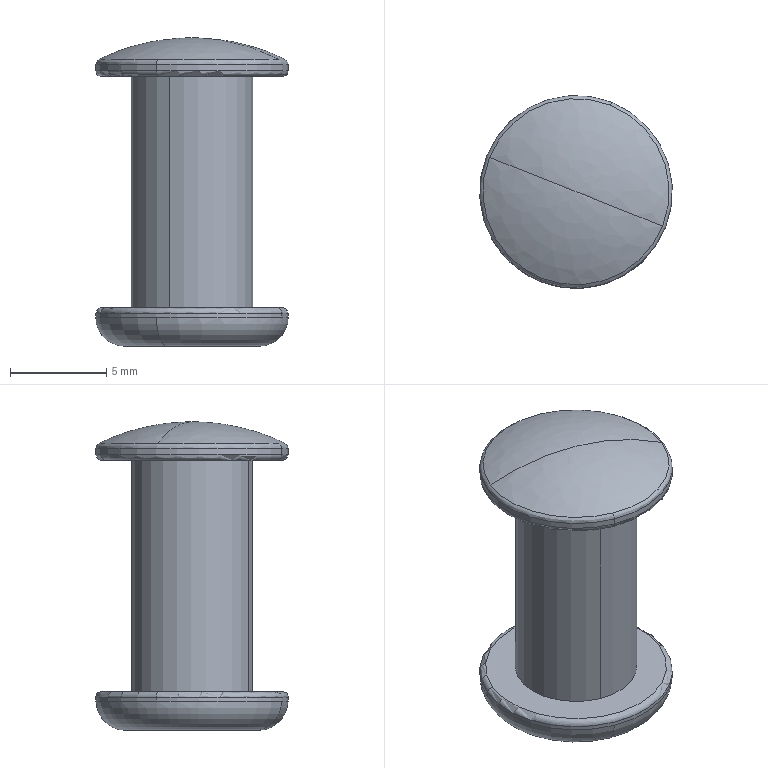Component | SolidWorks | CH-225-D-1_225-D-05-1 | 1 solid | 23 faces | box 10 x 10 x 16 mm | volume 564 mm3 | cylinder 8 | torus 6 | spline 4 | plane 3 | cone 2 | commonest cylinder face diameters 10 x4 6.3 x2 4.833 x2
STEP:
#1=COLOUR_RGB('',0.7922,0.8196,0.9333);
#2=FILL_AREA_STYLE_COLOUR('',#1);
#3=FILL_AREA_STYLE('',(#2));
#4=SURFACE_STYLE_FILL_AREA(#3);
#5=SURFACE_SIDE_STYLE('',(#4));
#6=SURFACE_STYLE_USAGE(.BOTH.,#5);
#7=PRESENTATION_STYLE_ASSIGNMENT((#6));
#8=CARTESIAN_POINT('',(0.9006,3.358,4.958));
#9=VERTEX_POINT('',#8);
#10=CARTESIAN_POINT('',(1.077,3.288,4.914));
#11=VERTEX_POINT('',#10);
#12=CARTESIAN_POINT('',(0.9006,3.358,4.525));
#13=DIRECTION('',(0.3691,0.9294,0.));
#14=DIRECTION('',(0.,0.,1.));
#15=AXIS2_PLACEMENT_3D('',#12,#13,#14);
#16=CIRCLE('',#15,0.4332);
#17=EDGE_CURVE('',#9,#11,#16,.T.);
#18=ORIENTED_EDGE('',*,*,#17,.F.);
#19=CARTESIAN_POINT('',(0.7238,3.429,4.914));
#20=VERTEX_POINT('',#19);
#21=CARTESIAN_POINT('',(0.9006,3.358,4.525));
#22=DIRECTION('',(-0.3691,-0.9294,0.));
#23=DIRECTION('',(0.,0.,1.));
#24=AXIS2_PLACEMENT_3D('',#21,#22,#23);
#25=CIRCLE('',#24,0.4332);
#26=EDGE_CURVE('',#9,#20,#25,.T.);
#27=ORIENTED_EDGE('',*,*,#26,.T.);
#28=CARTESIAN_POINT('',(0.8304,3.182,4.914));
#29=VERTEX_POINT('',#28);
#30=CARTESIAN_POINT('',(0.9006,3.358,4.914));
#31=DIRECTION('',(0.,0.,-1.));
#32=DIRECTION('',(0.3691,0.9294,0.));
#33=AXIS2_PLACEMENT_3D('',#30,#31,#32);
#34=CIRCLE('',#33,0.1902);
#35=EDGE_CURVE('',#29,#20,#34,.T.);
#36=ORIENTED_EDGE('',*,*,#35,.F.);
#37=CARTESIAN_POINT('',(0.9006,3.358,4.914));
#38=DIRECTION('',(0.,0.,-1.));
#39=DIRECTION('',(0.3691,0.9294,0.));
#40=AXIS2_PLACEMENT_3D('',#37,#38,#39);
#41=CIRCLE('',#40,0.1902);
#42=EDGE_CURVE('',#11,#29,#41,.T.);
#43=ORIENTED_EDGE('',*,*,#42,.F.);
#44=EDGE_LOOP('',(#18,#27,#36,#43));
#45=FACE_OUTER_BOUND('',#44,.T.);
#46=CARTESIAN_POINT('',(0.9006,3.358,4.958));
#47=CARTESIAN_POINT('',(0.9006,3.358,4.958));
#48=CARTESIAN_POINT('',(0.9006,3.358,4.958));
#49=CARTESIAN_POINT('',(0.9006,3.358,4.958));
#50=CARTESIAN_POINT('',(0.9622,3.334,4.958));
#51=CARTESIAN_POINT('',(0.9133,3.211,4.958));
#52=CARTESIAN_POINT('',(0.7902,3.26,4.958));
#53=CARTESIAN_POINT('',(0.8391,3.383,4.958));
#54=CARTESIAN_POINT('',(1.022,3.31,4.943));
#55=CARTESIAN_POINT('',(0.9256,3.067,4.943));
#56=CARTESIAN_POINT('',(0.6826,3.164,4.943));
#57=CARTESIAN_POINT('',(0.7791,3.407,4.943));
#58=CARTESIAN_POINT('',(1.077,3.288,4.914));
#59=CARTESIAN_POINT('',(0.937,2.935,4.914));
#60=CARTESIAN_POINT('',(0.5834,3.075,4.914));
#61=CARTESIAN_POINT('',(0.7238,3.429,4.914));
#62=(BOUNDED_SURFACE()B_SPLINE_SURFACE(3,3,((#46,#47,#48,#49),(#50,#51,#52,#53),(#54,#55,#56,#57),(#58,#59,#60,#61)),.UNSPECIFIED.,.F.,.F.,.F.)B_SPLINE_SURFACE_WITH_KNOTS((4,4),(4,4),(0.,1.),(0.,1.),.UNSPECIFIED.)GEOMETRIC_REPRESENTATION_ITEM()RATIONAL_B_SPLINE_SURFACE(((1.,0.3333,0.3333,1.),(0.9829,0.3276,0.3276,0.9829),(0.9829,0.3276,0.3276,0.9829),(1.,0.3333,0.3333,1.)))REPRESENTATION_ITEM('')SURFACE());
#63=ADVANCED_FACE('',(#45),#62,.F.);
#64=CARTESIAN_POINT('',(0.8548,3.243,4.879));
#65=VERTEX_POINT('',#64);
#66=CARTESIAN_POINT('',(0.9464,3.474,4.879));
#67=VERTEX_POINT('',#66);
#68=CARTESIAN_POINT('',(0.9006,3.358,4.879));
#69=DIRECTION('',(0.,0.,1.));
#70=DIRECTION('',(0.3691,0.9294,0.));
#71=AXIS2_PLACEMENT_3D('',#68,#69,#70);
#72=CIRCLE('',#71,0.124);
#73=EDGE_CURVE('',#65,#67,#72,.T.);
#74=ORIENTED_EDGE('',*,*,#73,.F.);
#75=CARTESIAN_POINT('',(0.8548,3.243,4.407));
#76=VERTEX_POINT('',#75);
#77=CARTESIAN_POINT('',(0.8548,3.243,4.879));
#78=DIRECTION('',(0.,0.,-1.));
#79=VECTOR('',#78,39.37);
#80=LINE('',#77,#79);
#81=EDGE_CURVE('',#65,#76,#80,.T.);
#82=ORIENTED_EDGE('',*,*,#81,.T.);
#83=CARTESIAN_POINT('',(0.9464,3.474,4.407));
#84=VERTEX_POINT('',#83);
#85=CARTESIAN_POINT('',(0.9006,3.358,4.407));
#86=DIRECTION('',(0.,0.,-1.));
#87=DIRECTION('',(0.3691,0.9294,0.));
#88=AXIS2_PLACEMENT_3D('',#85,#86,#87);
#89=CIRCLE('',#88,0.124);
#90=EDGE_CURVE('',#84,#76,#89,.T.);
#91=ORIENTED_EDGE('',*,*,#90,.F.);
#92=CARTESIAN_POINT('',(0.9464,3.474,4.879));
#93=DIRECTION('',(0.,0.,-1.));
#94=VECTOR('',#93,39.37);
#95=LINE('',#92,#94);
#96=EDGE_CURVE('',#67,#84,#95,.T.);
#97=ORIENTED_EDGE('',*,*,#96,.F.);
#98=EDGE_LOOP('',(#74,#82,#91,#97));
#99=FACE_OUTER_BOUND('',#98,.T.);
#100=CARTESIAN_POINT('',(0.9006,3.358,4.879));
#101=DIRECTION('',(0.,0.,-1.));
#102=DIRECTION('',(0.3691,0.9294,0.));
#103=AXIS2_PLACEMENT_3D('',#100,#101,#102);
#104=CYLINDRICAL_SURFACE('',#103,0.124);
#105=ADVANCED_FACE('',(#99),#104,.T.);
#106=CARTESIAN_POINT('',(0.9733,3.541,4.891));
#107=VERTEX_POINT('',#106);
#108=CARTESIAN_POINT('',(0.828,3.175,4.891));
#109=VERTEX_POINT('',#108);
#110=CARTESIAN_POINT('',(0.9006,3.358,4.891));
#111=DIRECTION('',(0.,0.,-1.));
#112=DIRECTION('',(0.3691,0.9294,0.));
#113=AXIS2_PLACEMENT_3D('',#110,#111,#112);
#114=CIRCLE('',#113,0.1969);
#115=EDGE_CURVE('',#107,#109,#114,.T.);
#116=ORIENTED_EDGE('',*,*,#115,.T.);
#117=CARTESIAN_POINT('',(0.8323,3.186,4.879));
#118=VERTEX_POINT('',#117);
#119=CARTESIAN_POINT('',(0.8323,3.186,4.891));
#120=DIRECTION('',(0.9294,-0.3691,0.));
#121=DIRECTION('',(0.3691,0.9294,0.));
#122=AXIS2_PLACEMENT_3D('',#119,#120,#121);
#123=CIRCLE('',#122,0.01181);
#124=EDGE_CURVE('',#109,#118,#123,.T.);
#125=ORIENTED_EDGE('',*,*,#124,.T.);
#126=CARTESIAN_POINT('',(0.9689,3.53,4.879));
#127=VERTEX_POINT('',#126);
#128=CARTESIAN_POINT('',(0.9006,3.358,4.879));
#129=DIRECTION('',(0.,0.,1.));
#130=DIRECTION('',(0.3691,0.9294,0.));
#131=AXIS2_PLACEMENT_3D('',#128,#129,#130);
#132=CIRCLE('',#131,0.185);
#133=EDGE_CURVE('',#118,#127,#132,.T.);
#134=ORIENTED_EDGE('',*,*,#133,.T.);
#135=CARTESIAN_POINT('',(0.9689,3.53,4.891));
#136=DIRECTION('',(-0.9294,0.3691,0.));
#137=DIRECTION('',(-0.3691,-0.9294,0.));
#138=AXIS2_PLACEMENT_3D('',#135,#136,#137);
#139=CIRCLE('',#138,0.01181);
#140=EDGE_CURVE('',#107,#127,#139,.T.);
#141=ORIENTED_EDGE('',*,*,#140,.F.);
#142=EDGE_LOOP('',(#116,#125,#134,#141));
#143=FACE_OUTER_BOUND('',#142,.T.);
#144=CARTESIAN_POINT('',(0.9006,3.358,4.891));
#145=DIRECTION('',(0.,0.,-1.));
#146=DIRECTION('',(0.3691,0.9294,0.));
#147=AXIS2_PLACEMENT_3D('',#144,#145,#146);
#148=TOROIDAL_SURFACE('',#147,0.185,0.01181);
#149=ADVANCED_FACE('',(#143),#148,.T.);
#150=CARTESIAN_POINT('',(0.7286,3.427,4.407));
#151=VERTEX_POINT('',#150);
#152=CARTESIAN_POINT('',(1.073,3.29,4.407));
#153=VERTEX_POINT('',#152);
#154=CARTESIAN_POINT('',(0.9006,3.358,4.407));
#155=DIRECTION('',(0.,-0.,-1.));
#156=DIRECTION('',(-0.9294,0.3691,0.));
#157=AXIS2_PLACEMENT_3D('',#154,#155,#156);
#158=CIRCLE('',#157,0.185);
#159=EDGE_CURVE('',#151,#153,#158,.T.);
#160=ORIENTED_EDGE('',*,*,#159,.T.);
#161=CARTESIAN_POINT('',(1.084,3.286,4.395));
#162=VERTEX_POINT('',#161);
#163=CARTESIAN_POINT('',(1.073,3.29,4.395));
#164=DIRECTION('',(0.3691,0.9294,-0.));
#165=DIRECTION('',(-0.9294,0.3691,0.));
#166=AXIS2_PLACEMENT_3D('',#163,#164,#165);
#167=CIRCLE('',#166,0.01181);
#168=EDGE_CURVE('',#153,#162,#167,.T.);
#169=ORIENTED_EDGE('',*,*,#168,.T.);
#170=CARTESIAN_POINT('',(0.7177,3.431,4.395));
#171=VERTEX_POINT('',#170);
#172=CARTESIAN_POINT('',(0.9006,3.358,4.395));
#173=DIRECTION('',(-0.,0.,1.));
#174=DIRECTION('',(0.9294,-0.3691,0.));
#175=AXIS2_PLACEMENT_3D('',#172,#173,#174);
#176=CIRCLE('',#175,0.1969);
#177=EDGE_CURVE('',#162,#171,#176,.T.);
#178=ORIENTED_EDGE('',*,*,#177,.T.);
#179=CARTESIAN_POINT('',(0.7286,3.427,4.395));
#180=DIRECTION('',(-0.3691,-0.9294,0.));
#181=DIRECTION('',(0.9294,-0.3691,0.));
#182=AXIS2_PLACEMENT_3D('',#179,#180,#181);
#183=CIRCLE('',#182,0.01181);
#184=EDGE_CURVE('',#151,#171,#183,.T.);
#185=ORIENTED_EDGE('',*,*,#184,.F.);
#186=EDGE_LOOP('',(#160,#169,#178,#185));
#187=FACE_OUTER_BOUND('',#186,.T.);
#188=CARTESIAN_POINT('',(0.9006,3.358,4.395));
#189=DIRECTION('',(0.,-0.,-1.));
#190=DIRECTION('',(-0.9294,0.3691,-0.));
#191=AXIS2_PLACEMENT_3D('',#188,#189,#190);
#192=TOROIDAL_SURFACE('',#191,0.185,0.01181);
#193=ADVANCED_FACE('',(#187),#192,.T.);
#194=CARTESIAN_POINT('',(0.828,3.175,4.903));
#195=VERTEX_POINT('',#194);
#196=CARTESIAN_POINT('',(0.9733,3.541,4.903));
#197=VERTEX_POINT('',#196);
#198=CARTESIAN_POINT('',(0.9006,3.358,4.903));
#199=DIRECTION('',(0.,0.,1.));
#200=DIRECTION('',(0.3691,0.9294,0.));
#201=AXIS2_PLACEMENT_3D('',#198,#199,#200);
#202=CIRCLE('',#201,0.1969);
#203=EDGE_CURVE('',#195,#197,#202,.T.);
#204=ORIENTED_EDGE('',*,*,#203,.F.);
#205=CARTESIAN_POINT('',(0.828,3.175,4.903));
#206=DIRECTION('',(0.,0.,-1.));
#207=VECTOR('',#206,39.37);
#208=LINE('',#205,#207);
#209=EDGE_CURVE('',#195,#109,#208,.T.);
#210=ORIENTED_EDGE('',*,*,#209,.T.);
#211=ORIENTED_EDGE('',*,*,#115,.F.);
#212=CARTESIAN_POINT('',(0.9733,3.541,4.903));
#213=DIRECTION('',(0.,0.,-1.));
#214=VECTOR('',#213,39.37);
#215=LINE('',#212,#214);
#216=EDGE_CURVE('',#197,#107,#215,.T.);
#217=ORIENTED_EDGE('',*,*,#216,.F.);
#218=EDGE_LOOP('',(#204,#210,#211,#217));
#219=FACE_OUTER_BOUND('',#218,.T.);
#220=CARTESIAN_POINT('',(0.9006,3.358,4.903));
#221=DIRECTION('',(0.,0.,-1.));
#222=DIRECTION('',(0.3691,0.9294,0.));
#223=AXIS2_PLACEMENT_3D('',#220,#221,#222);
#224=CYLINDRICAL_SURFACE('',#223,0.1969);
#225=ADVANCED_FACE('',(#219),#224,.T.);
#226=ORIENTED_EDGE('',*,*,#177,.F.);
#227=CARTESIAN_POINT('',(1.084,3.286,4.387));
#228=VERTEX_POINT('',#227);
#229=CARTESIAN_POINT('',(1.084,3.286,4.395));
#230=DIRECTION('',(0.,-0.,-1.));
#231=VECTOR('',#230,39.37);
#232=LINE('',#229,#231);
#233=EDGE_CURVE('',#162,#228,#232,.T.);
#234=ORIENTED_EDGE('',*,*,#233,.T.);
#235=CARTESIAN_POINT('',(0.9733,3.541,4.387));
#236=VERTEX_POINT('',#235);
#237=CARTESIAN_POINT('',(0.9006,3.358,4.387));
#238=DIRECTION('',(0.,0.,-1.));
#239=DIRECTION('',(0.3691,0.9294,0.));
#240=AXIS2_PLACEMENT_3D('',#237,#238,#239);
#241=CIRCLE('',#240,0.1969);
#242=EDGE_CURVE('',#236,#228,#241,.T.);
#243=ORIENTED_EDGE('',*,*,#242,.F.);
#244=CARTESIAN_POINT('',(0.7177,3.431,4.387));
#245=VERTEX_POINT('',#244);
#246=CARTESIAN_POINT('',(0.9006,3.358,4.387));
#247=DIRECTION('',(0.,0.,-1.));
#248=DIRECTION('',(0.3691,0.9294,0.));
#249=AXIS2_PLACEMENT_3D('',#246,#247,#248);
#250=CIRCLE('',#249,0.1969);
#251=EDGE_CURVE('',#245,#236,#250,.T.);
#252=ORIENTED_EDGE('',*,*,#251,.F.);
#253=CARTESIAN_POINT('',(0.7177,3.431,4.395));
#254=DIRECTION('',(0.,-0.,-1.));
#255=VECTOR('',#254,39.37);
#256=LINE('',#253,#255);
#257=EDGE_CURVE('',#171,#245,#256,.T.);
#258=ORIENTED_EDGE('',*,*,#257,.F.);
#259=EDGE_LOOP('',(#226,#234,#243,#252,#258));
#260=FACE_OUTER_BOUND('',#259,.T.);
#261=CARTESIAN_POINT('',(0.9006,3.358,4.395));
#262=DIRECTION('',(0.,-0.,-1.));
#263=DIRECTION('',(-0.9294,0.3691,0.));
#264=AXIS2_PLACEMENT_3D('',#261,#262,#263);
#265=CYLINDRICAL_SURFACE('',#264,0.1969);
#266=ADVANCED_FACE('',(#260),#265,.T.);
#267=ORIENTED_EDGE('',*,*,#242,.T.);
#268=CARTESIAN_POINT('',(0.828,3.175,4.387));
#269=VERTEX_POINT('',#268);
#270=CARTESIAN_POINT('',(0.9006,3.358,4.387));
#271=DIRECTION('',(0.,0.,-1.));
#272=DIRECTION('',(0.3691,0.9294,0.));
#273=AXIS2_PLACEMENT_3D('',#270,#271,#272);
#274=CIRCLE('',#273,0.1969);
#275=EDGE_CURVE('',#228,#269,#274,.T.);
#276=ORIENTED_EDGE('',*,*,#275,.T.);
#277=CARTESIAN_POINT('',(0.8498,3.23,4.328));
#278=VERTEX_POINT('',#277);
#279=CARTESIAN_POINT('',(0.8498,3.23,4.387));
#280=DIRECTION('',(0.9294,-0.3691,0.));
#281=DIRECTION('',(0.3691,0.9294,0.));
#282=AXIS2_PLACEMENT_3D('',#279,#280,#281);
#283=CIRCLE('',#282,0.05906);
#284=EDGE_CURVE('',#269,#278,#283,.T.);
#285=ORIENTED_EDGE('',*,*,#284,.T.);
#286=CARTESIAN_POINT('',(0.9515,3.486,4.328));
#287=VERTEX_POINT('',#286);
#288=CARTESIAN_POINT('',(0.9006,3.358,4.328));
#289=DIRECTION('',(0.,0.,1.));
#290=DIRECTION('',(0.3691,0.9294,0.));
#291=AXIS2_PLACEMENT_3D('',#288,#289,#290);
#292=CIRCLE('',#291,0.1378);
#293=EDGE_CURVE('',#278,#287,#292,.T.);
#294=ORIENTED_EDGE('',*,*,#293,.T.);
#295=CARTESIAN_POINT('',(0.9515,3.486,4.387));
#296=DIRECTION('',(-0.9294,0.3691,0.));
#297=DIRECTION('',(-0.3691,-0.9294,0.));
#298=AXIS2_PLACEMENT_3D('',#295,#296,#297);
#299=CIRCLE('',#298,0.05906);
#300=EDGE_CURVE('',#236,#287,#299,.T.);
#301=ORIENTED_EDGE('',*,*,#300,.F.);
#302=EDGE_LOOP('',(#267,#276,#285,#294,#301));
#303=FACE_OUTER_BOUND('',#302,.T.);
#304=CARTESIAN_POINT('',(0.9006,3.358,4.387));
#305=DIRECTION('',(0.,0.,-1.));
#306=DIRECTION('',(0.3691,0.9294,0.));
#307=AXIS2_PLACEMENT_3D('',#304,#305,#306);
#308=TOROIDAL_SURFACE('',#307,0.1378,0.05906);
#309=ADVANCED_FACE('',(#303),#308,.T.);
#310=CARTESIAN_POINT('',(0.9357,3.447,4.446));
#311=VERTEX_POINT('',#310);
#312=CARTESIAN_POINT('',(0.8655,3.27,4.446));
#313=VERTEX_POINT('',#312);
#314=CARTESIAN_POINT('',(0.9006,3.358,4.446));
#315=DIRECTION('',(0.,0.,1.));
#316=DIRECTION('',(0.3691,0.9294,0.));
#317=AXIS2_PLACEMENT_3D('',#314,#315,#316);
#318=CIRCLE('',#317,0.09515);
#319=EDGE_CURVE('',#311,#313,#318,.T.);
#320=ORIENTED_EDGE('',*,*,#319,.T.);
#321=CARTESIAN_POINT('',(0.8655,3.27,4.328));
#322=VERTEX_POINT('',#321);
#323=CARTESIAN_POINT('',(0.8655,3.27,4.446));
#324=DIRECTION('',(0.,0.,-1.));
#325=VECTOR('',#324,39.37);
#326=LINE('',#323,#325);
#327=EDGE_CURVE('',#313,#322,#326,.T.);
#328=ORIENTED_EDGE('',*,*,#327,.T.);
#329=CARTESIAN_POINT('',(0.9357,3.447,4.328));
#330=VERTEX_POINT('',#329);
#331=CARTESIAN_POINT('',(0.9006,3.358,4.328));
#332=DIRECTION('',(0.,0.,-1.));
#333=DIRECTION('',(0.3691,0.9294,0.));
#334=AXIS2_PLACEMENT_3D('',#331,#332,#333);
#335=CIRCLE('',#334,0.09515);
#336=EDGE_CURVE('',#322,#330,#335,.T.);
#337=ORIENTED_EDGE('',*,*,#336,.T.);
#338=CARTESIAN_POINT('',(0.9357,3.447,4.446));
#339=DIRECTION('',(0.,0.,-1.));
#340=VECTOR('',#339,39.37);
#341=LINE('',#338,#340);
#342=EDGE_CURVE('',#311,#330,#341,.T.);
#343=ORIENTED_EDGE('',*,*,#342,.F.);
#344=EDGE_LOOP('',(#320,#328,#337,#343));
#345=FACE_OUTER_BOUND('',#344,.T.);
#346=CARTESIAN_POINT('',(0.9006,3.358,4.446));
#347=DIRECTION('',(0.,0.,-1.));
#348=DIRECTION('',(0.3691,0.9294,0.));
#349=AXIS2_PLACEMENT_3D('',#346,#347,#348);
#350=CYLINDRICAL_SURFACE('',#349,0.09515);
#351=ADVANCED_FACE('',(#345),#350,.F.);
#352=CARTESIAN_POINT('',(0.9006,3.358,4.493));
#353=VERTEX_POINT('',#352);
#354=CARTESIAN_POINT('',(0.9006,3.358,4.493));
#355=DIRECTION('',(0.3306,0.8324,-0.4447));
#356=VECTOR('',#355,39.37);
#357=LINE('',#354,#356);
#358=EDGE_CURVE('',#353,#311,#357,.T.);
#359=ORIENTED_EDGE('',*,*,#358,.F.);
#360=CARTESIAN_POINT('',(0.9006,3.358,4.493));
#361=DIRECTION('',(-0.3306,-0.8324,-0.4447));
#362=VECTOR('',#361,39.37);
#363=LINE('',#360,#362);
#364=EDGE_CURVE('',#353,#313,#363,.T.);
#365=ORIENTED_EDGE('',*,*,#364,.T.);
#366=ORIENTED_EDGE('',*,*,#319,.F.);
#367=EDGE_LOOP('',(#359,#365,#366));
#368=FACE_OUTER_BOUND('',#367,.T.);
#369=CARTESIAN_POINT('',(0.9006,3.358,-34.877));
#370=DIRECTION('',(0.,0.,-1.));
#371=DIRECTION('',(0.3691,0.9294,0.));
#372=AXIS2_PLACEMENT_3D('',#369,#370,#371);
#373=CONICAL_SURFACE('',#372,79.288,1.11);
#374=ADVANCED_FACE('',(#368),#373,.F.);
#375=ORIENTED_EDGE('',*,*,#81,.F.);
#376=CARTESIAN_POINT('',(0.9006,3.358,4.879));
#377=DIRECTION('',(0.,0.,1.));
#378=DIRECTION('',(0.3691,0.9294,0.));
#379=AXIS2_PLACEMENT_3D('',#376,#377,#378);
#380=CIRCLE('',#379,0.124);
#381=EDGE_CURVE('',#67,#65,#380,.T.);
#382=ORIENTED_EDGE('',*,*,#381,.F.);
#383=ORIENTED_EDGE('',*,*,#96,.T.);
#384=CARTESIAN_POINT('',(0.9006,3.358,4.407));
#385=DIRECTION('',(0.,0.,-1.));
#386=DIRECTION('',(0.3691,0.9294,0.));
#387=AXIS2_PLACEMENT_3D('',#384,#385,#386);
#388=CIRCLE('',#387,0.124);
#389=EDGE_CURVE('',#76,#84,#388,.T.);
#390=ORIENTED_EDGE('',*,*,#389,.F.);
#391=EDGE_LOOP('',(#375,#382,#383,#390));
#392=FACE_OUTER_BOUND('',#391,.T.);
#393=CARTESIAN_POINT('',(0.9006,3.358,4.879));
#394=DIRECTION('',(0.,0.,-1.));
#395=DIRECTION('',(0.3691,0.9294,0.));
#396=AXIS2_PLACEMENT_3D('',#393,#394,#395);
#397=CYLINDRICAL_SURFACE('',#396,0.124);
#398=ADVANCED_FACE('',(#392),#397,.T.);
#399=ORIENTED_EDGE('',*,*,#381,.T.);
#400=ORIENTED_EDGE('',*,*,#73,.T.);
#401=EDGE_LOOP('',(#399,#400));
#402=FACE_BOUND('',#401,.T.);
#403=CARTESIAN_POINT('',(0.9006,3.358,4.879));
#404=DIRECTION('',(0.,0.,1.));
#405=DIRECTION('',(0.3691,0.9294,0.));
#406=AXIS2_PLACEMENT_3D('',#403,#404,#405);
#407=CIRCLE('',#406,0.185);
#408=EDGE_CURVE('',#127,#118,#407,.T.);
#409=ORIENTED_EDGE('',*,*,#408,.F.);
#410=ORIENTED_EDGE('',*,*,#133,.F.);
#411=EDGE_LOOP('',(#409,#410));
#412=FACE_OUTER_BOUND('',#411,.T.);
#413=CARTESIAN_POINT('',(0.7957,3.601,4.879));
#414=DIRECTION('',(0.,0.,1.));
#415=DIRECTION('',(-0.3691,-0.9294,0.));
#416=AXIS2_PLACEMENT_3D('',#413,#414,#415);
#417=PLANE('',#416);
#418=ADVANCED_FACE('',(#402,#412),#417,.F.);
#419=ORIENTED_EDGE('',*,*,#90,.T.);
#420=ORIENTED_EDGE('',*,*,#389,.T.);
#421=EDGE_LOOP('',(#419,#420));
#422=FACE_BOUND('',#421,.T.);
#423=ORIENTED_EDGE('',*,*,#159,.F.);
#424=CARTESIAN_POINT('',(0.9006,3.358,4.407));
#425=DIRECTION('',(0.,-0.,-1.));
#426=DIRECTION('',(-0.9294,0.3691,0.));
#427=AXIS2_PLACEMENT_3D('',#424,#425,#426);
#428=CIRCLE('',#427,0.185);
#429=EDGE_CURVE('',#153,#151,#428,.T.);
#430=ORIENTED_EDGE('',*,*,#429,.F.);
#431=EDGE_LOOP('',(#423,#430));
#432=FACE_OUTER_BOUND('',#431,.T.);
#433=CARTESIAN_POINT('',(0.6575,3.253,4.407));
#434=DIRECTION('',(0.,0.,-1.));
#435=DIRECTION('',(0.3691,0.9294,0.));
#436=AXIS2_PLACEMENT_3D('',#433,#434,#435);
#437=PLANE('',#436);
#438=ADVANCED_FACE('',(#422,#432),#437,.F.);
#439=ORIENTED_EDGE('',*,*,#124,.F.);
#440=CARTESIAN_POINT('',(0.9006,3.358,4.891));
#441=DIRECTION('',(0.,0.,-1.));
#442=DIRECTION('',(0.3691,0.9294,0.));
#443=AXIS2_PLACEMENT_3D('',#440,#441,#442);
#444=CIRCLE('',#443,0.1969);
#445=EDGE_CURVE('',#109,#107,#444,.T.);
#446=ORIENTED_EDGE('',*,*,#445,.T.);
#447=ORIENTED_EDGE('',*,*,#140,.T.);
#448=ORIENTED_EDGE('',*,*,#408,.T.);
#449=EDGE_LOOP('',(#439,#446,#447,#448));
#450=FACE_OUTER_BOUND('',#449,.T.);
#451=CARTESIAN_POINT('',(0.9006,3.358,4.891));
#452=DIRECTION('',(0.,0.,-1.));
#453=DIRECTION('',(0.3691,0.9294,0.));
#454=AXIS2_PLACEMENT_3D('',#451,#452,#453);
#455=TOROIDAL_SURFACE('',#454,0.185,0.01181);
#456=ADVANCED_FACE('',(#450),#455,.T.);
#457=ORIENTED_EDGE('',*,*,#168,.F.);
#458=ORIENTED_EDGE('',*,*,#429,.T.);
#459=ORIENTED_EDGE('',*,*,#184,.T.);
#460=CARTESIAN_POINT('',(0.9006,3.358,4.395));
#461=DIRECTION('',(-0.,0.,1.));
#462=DIRECTION('',(0.9294,-0.3691,0.));
#463=AXIS2_PLACEMENT_3D('',#460,#461,#462);
#464=CIRCLE('',#463,0.1969);
#465=EDGE_CURVE('',#171,#162,#464,.T.);
#466=ORIENTED_EDGE('',*,*,#465,.T.);
#467=EDGE_LOOP('',(#457,#458,#459,#466));
#468=FACE_OUTER_BOUND('',#467,.T.);
#469=CARTESIAN_POINT('',(0.9006,3.358,4.395));
#470=DIRECTION('',(0.,-0.,-1.));
#471=DIRECTION('',(-0.9294,0.3691,-0.));
#472=AXIS2_PLACEMENT_3D('',#469,#470,#471);
#473=TOROIDAL_SURFACE('',#472,0.185,0.01181);
#474=ADVANCED_FACE('',(#468),#473,.T.);
#475=ORIENTED_EDGE('',*,*,#209,.F.);
#476=CARTESIAN_POINT('',(0.9006,3.358,4.903));
#477=DIRECTION('',(0.,0.,1.));
#478=DIRECTION('',(0.3691,0.9294,0.));
#479=AXIS2_PLACEMENT_3D('',#476,#477,#478);
#480=CIRCLE('',#479,0.1969);
#481=EDGE_CURVE('',#197,#195,#480,.T.);
#482=ORIENTED_EDGE('',*,*,#481,.F.);
#483=ORIENTED_EDGE('',*,*,#216,.T.);
#484=ORIENTED_EDGE('',*,*,#445,.F.);
#485=EDGE_LOOP('',(#475,#482,#483,#484));
#486=FACE_OUTER_BOUND('',#485,.T.);
#487=CARTESIAN_POINT('',(0.9006,3.358,4.903));
#488=DIRECTION('',(0.,0.,-1.));
#489=DIRECTION('',(0.3691,0.9294,0.));
#490=AXIS2_PLACEMENT_3D('',#487,#488,#489);
#491=CYLINDRICAL_SURFACE('',#490,0.1969);
#492=ADVANCED_FACE('',(#486),#491,.T.);
#493=ORIENTED_EDGE('',*,*,#233,.F.);
#494=ORIENTED_EDGE('',*,*,#465,.F.);
#495=ORIENTED_EDGE('',*,*,#257,.T.);
#496=CARTESIAN_POINT('',(0.9006,3.358,4.387));
#497=DIRECTION('',(0.,0.,-1.));
#498=DIRECTION('',(0.3691,0.9294,0.));
#499=AXIS2_PLACEMENT_3D('',#496,#497,#498);
#500=CIRCLE('',#499,0.1969);
#501=EDGE_CURVE('',#269,#245,#500,.T.);
#502=ORIENTED_EDGE('',*,*,#501,.F.);
#503=ORIENTED_EDGE('',*,*,#275,.F.);
#504=EDGE_LOOP('',(#493,#494,#495,#502,#503));
#505=FACE_OUTER_BOUND('',#504,.T.);
#506=CARTESIAN_POINT('',(0.9006,3.358,4.395));
#507=DIRECTION('',(0.,-0.,-1.));
#508=DIRECTION('',(-0.9294,0.3691,0.));
#509=AXIS2_PLACEMENT_3D('',#506,#507,#508);
#510=CYLINDRICAL_SURFACE('',#509,0.1969);
#511=ADVANCED_FACE('',(#505),#510,.T.);
#512=ORIENTED_EDGE('',*,*,#203,.T.);
#513=CARTESIAN_POINT('',(0.9708,3.535,4.914));
#514=VERTEX_POINT('',#513);
#515=CARTESIAN_POINT('',(0.9733,3.541,4.903));
#516=CARTESIAN_POINT('',(0.9733,3.541,4.908));
#517=CARTESIAN_POINT('',(0.9724,3.539,4.912));
#518=CARTESIAN_POINT('',(0.9708,3.535,4.914));
#519=(BOUNDED_CURVE()B_SPLINE_CURVE(3,(#515,#516,#517,#518),.UNSPECIFIED.,.F.,.F.)B_SPLINE_CURVE_WITH_KNOTS((4,4),(0.,1.),.UNSPECIFIED.)CURVE()GEOMETRIC_REPRESENTATION_ITEM()RATIONAL_B_SPLINE_CURVE((1.,0.8988,0.8988,1.))REPRESENTATION_ITEM(''));
#520=EDGE_CURVE('',#197,#514,#519,.T.);
#521=ORIENTED_EDGE('',*,*,#520,.T.);
#522=CARTESIAN_POINT('',(0.9006,3.358,4.914));
#523=DIRECTION('',(0.,0.,-1.));
#524=DIRECTION('',(0.3691,0.9294,0.));
#525=AXIS2_PLACEMENT_3D('',#522,#523,#524);
#526=CIRCLE('',#525,0.1902);
#527=EDGE_CURVE('',#514,#11,#526,.T.);
#528=ORIENTED_EDGE('',*,*,#527,.T.);
#529=ORIENTED_EDGE('',*,*,#42,.T.);
#530=CARTESIAN_POINT('',(0.8304,3.182,4.914));
#531=CARTESIAN_POINT('',(0.8289,3.178,4.912));
#532=CARTESIAN_POINT('',(0.828,3.175,4.908));
#533=CARTESIAN_POINT('',(0.828,3.175,4.903));
#534=(BOUNDED_CURVE()B_SPLINE_CURVE(3,(#530,#531,#532,#533),.UNSPECIFIED.,.F.,.F.)B_SPLINE_CURVE_WITH_KNOTS((4,4),(0.,1.),.UNSPECIFIED.)CURVE()GEOMETRIC_REPRESENTATION_ITEM()RATIONAL_B_SPLINE_CURVE((1.,0.8988,0.8988,1.))REPRESENTATION_ITEM(''));
#535=EDGE_CURVE('',#29,#195,#534,.T.);
#536=ORIENTED_EDGE('',*,*,#535,.T.);
#537=EDGE_LOOP('',(#512,#521,#528,#529,#536));
#538=FACE_OUTER_BOUND('',#537,.T.);
#539=CARTESIAN_POINT('',(0.9733,3.541,4.903));
#540=CARTESIAN_POINT('',(1.339,3.396,4.903));
#541=CARTESIAN_POINT('',(1.194,3.03,4.903));
#542=CARTESIAN_POINT('',(0.828,3.175,4.903));
#543=CARTESIAN_POINT('',(0.9733,3.541,4.908));
#544=CARTESIAN_POINT('',(1.339,3.396,4.908));
#545=CARTESIAN_POINT('',(1.194,3.03,4.908));
#546=CARTESIAN_POINT('',(0.828,3.175,4.908));
#547=CARTESIAN_POINT('',(0.9724,3.539,4.912));
#548=CARTESIAN_POINT('',(1.334,3.395,4.912));
#549=CARTESIAN_POINT('',(1.19,3.034,4.912));
#550=CARTESIAN_POINT('',(0.8289,3.178,4.912));
#551=CARTESIAN_POINT('',(0.9708,3.535,4.914));
#552=CARTESIAN_POINT('',(1.324,3.395,4.914));
#553=CARTESIAN_POINT('',(1.184,3.041,4.914));
#554=CARTESIAN_POINT('',(0.8304,3.182,4.914));
#555=(BOUNDED_SURFACE()B_SPLINE_SURFACE(3,3,((#539,#540,#541,#542),(#543,#544,#545,#546),(#547,#548,#549,#550),(#551,#552,#553,#554)),.UNSPECIFIED.,.F.,.F.,.F.)B_SPLINE_SURFACE_WITH_KNOTS((4,4),(4,4),(0.,1.),(0.,1.),.UNSPECIFIED.)GEOMETRIC_REPRESENTATION_ITEM()RATIONAL_B_SPLINE_SURFACE(((1.,0.3333,0.3333,1.),(0.8988,0.2996,0.2996,0.8988),(0.8988,0.2996,0.2996,0.8988),(1.,0.3333,0.3333,1.)))REPRESENTATION_ITEM('')SURFACE());
#556=ADVANCED_FACE('',(#538),#555,.T.);
#557=ORIENTED_EDGE('',*,*,#520,.F.);
#558=ORIENTED_EDGE('',*,*,#481,.T.);
#559=ORIENTED_EDGE('',*,*,#535,.F.);
#560=ORIENTED_EDGE('',*,*,#35,.T.);
#561=CARTESIAN_POINT('',(0.9006,3.358,4.914));
#562=DIRECTION('',(0.,0.,-1.));
#563=DIRECTION('',(0.3691,0.9294,0.));
#564=AXIS2_PLACEMENT_3D('',#561,#562,#563);
#565=CIRCLE('',#564,0.1902);
#566=EDGE_CURVE('',#20,#514,#565,.T.);
#567=ORIENTED_EDGE('',*,*,#566,.T.);
#568=EDGE_LOOP('',(#557,#558,#559,#560,#567));
#569=FACE_OUTER_BOUND('',#568,.T.);
#570=CARTESIAN_POINT('',(0.828,3.175,4.903));
#571=CARTESIAN_POINT('',(0.4621,3.321,4.903));
#572=CARTESIAN_POINT('',(0.6074,3.687,4.903));
#573=CARTESIAN_POINT('',(0.9733,3.541,4.903));
#574=CARTESIAN_POINT('',(0.828,3.175,4.908));
#575=CARTESIAN_POINT('',(0.4621,3.321,4.908));
#576=CARTESIAN_POINT('',(0.6074,3.687,4.908));
#577=CARTESIAN_POINT('',(0.9733,3.541,4.908));
#578=CARTESIAN_POINT('',(0.8289,3.178,4.912));
#579=CARTESIAN_POINT('',(0.4675,3.321,4.912));
#580=CARTESIAN_POINT('',(0.611,3.682,4.912));
#581=CARTESIAN_POINT('',(0.9724,3.539,4.912));
#582=CARTESIAN_POINT('',(0.8304,3.182,4.914));
#583=CARTESIAN_POINT('',(0.4768,3.322,4.914));
#584=CARTESIAN_POINT('',(0.6172,3.676,4.914));
#585=CARTESIAN_POINT('',(0.9708,3.535,4.914));
#586=(BOUNDED_SURFACE()B_SPLINE_SURFACE(3,3,((#570,#571,#572,#573),(#574,#575,#576,#577),(#578,#579,#580,#581),(#582,#583,#584,#585)),.UNSPECIFIED.,.F.,.F.,.F.)B_SPLINE_SURFACE_WITH_KNOTS((4,4),(4,4),(0.,1.),(0.,1.),.UNSPECIFIED.)GEOMETRIC_REPRESENTATION_ITEM()RATIONAL_B_SPLINE_SURFACE(((1.,0.3333,0.3333,1.),(0.8988,0.2996,0.2996,0.8988),(0.8988,0.2996,0.2996,0.8988),(1.,0.3333,0.3333,1.)))REPRESENTATION_ITEM('')SURFACE());
#587=ADVANCED_FACE('',(#569),#586,.T.);
#588=ORIENTED_EDGE('',*,*,#284,.F.);
#589=ORIENTED_EDGE('',*,*,#501,.T.);
#590=ORIENTED_EDGE('',*,*,#251,.T.);
#591=ORIENTED_EDGE('',*,*,#300,.T.);
#592=CARTESIAN_POINT('',(0.9006,3.358,4.328));
#593=DIRECTION('',(0.,0.,1.));
#594=DIRECTION('',(0.3691,0.9294,0.));
#595=AXIS2_PLACEMENT_3D('',#592,#593,#594);
#596=CIRCLE('',#595,0.1378);
#597=EDGE_CURVE('',#287,#278,#596,.T.);
#598=ORIENTED_EDGE('',*,*,#597,.T.);
#599=EDGE_LOOP('',(#588,#589,#590,#591,#598));
#600=FACE_OUTER_BOUND('',#599,.T.);
#601=CARTESIAN_POINT('',(0.9006,3.358,4.387));
#602=DIRECTION('',(0.,0.,-1.));
#603=DIRECTION('',(0.3691,0.9294,0.));
#604=AXIS2_PLACEMENT_3D('',#601,#602,#603);
#605=TOROIDAL_SURFACE('',#604,0.1378,0.05906);
#606=ADVANCED_FACE('',(#600),#605,.T.);
#607=ORIENTED_EDGE('',*,*,#26,.F.);
#608=ORIENTED_EDGE('',*,*,#17,.T.);
#609=ORIENTED_EDGE('',*,*,#527,.F.);
#610=ORIENTED_EDGE('',*,*,#566,.F.);
#611=EDGE_LOOP('',(#607,#608,#609,#610));
#612=FACE_OUTER_BOUND('',#611,.T.);
#613=CARTESIAN_POINT('',(0.9006,3.358,4.958));
#614=CARTESIAN_POINT('',(0.9006,3.358,4.958));
#615=CARTESIAN_POINT('',(0.9006,3.358,4.958));
#616=CARTESIAN_POINT('',(0.9006,3.358,4.958));
#617=CARTESIAN_POINT('',(0.8391,3.383,4.958));
#618=CARTESIAN_POINT('',(0.888,3.506,4.958));
#619=CARTESIAN_POINT('',(1.011,3.457,4.958));
#620=CARTESIAN_POINT('',(0.9622,3.334,4.958));
#621=CARTESIAN_POINT('',(0.7791,3.407,4.943));
#622=CARTESIAN_POINT('',(0.8756,3.65,4.943));
#623=CARTESIAN_POINT('',(1.119,3.553,4.943));
#624=CARTESIAN_POINT('',(1.022,3.31,4.943));
#625=CARTESIAN_POINT('',(0.7238,3.429,4.914));
#626=CARTESIAN_POINT('',(0.8642,3.782,4.914));
#627=CARTESIAN_POINT('',(1.218,3.642,4.914));
#628=CARTESIAN_POINT('',(1.077,3.288,4.914));
#629=(BOUNDED_SURFACE()B_SPLINE_SURFACE(3,3,((#613,#614,#615,#616),(#617,#618,#619,#620),(#621,#622,#623,#624),(#625,#626,#627,#628)),.UNSPECIFIED.,.F.,.F.,.F.)B_SPLINE_SURFACE_WITH_KNOTS((4,4),(4,4),(0.,1.),(0.,1.),.UNSPECIFIED.)GEOMETRIC_REPRESENTATION_ITEM()RATIONAL_B_SPLINE_SURFACE(((1.,0.3333,0.3333,1.),(0.9829,0.3276,0.3276,0.9829),(0.9829,0.3276,0.3276,0.9829),(1.,0.3333,0.3333,1.)))REPRESENTATION_ITEM('')SURFACE());
#630=ADVANCED_FACE('',(#612),#629,.F.);
#631=CARTESIAN_POINT('',(0.9006,3.358,4.328));
#632=DIRECTION('',(0.,0.,-1.));
#633=DIRECTION('',(0.3691,0.9294,0.));
#634=AXIS2_PLACEMENT_3D('',#631,#632,#633);
#635=CIRCLE('',#634,0.09515);
#636=EDGE_CURVE('',#330,#322,#635,.T.);
#637=ORIENTED_EDGE('',*,*,#636,.F.);
#638=ORIENTED_EDGE('',*,*,#336,.F.);
#639=EDGE_LOOP('',(#637,#638));
#640=FACE_BOUND('',#639,.T.);
#641=ORIENTED_EDGE('',*,*,#597,.F.);
#642=ORIENTED_EDGE('',*,*,#293,.F.);
#643=EDGE_LOOP('',(#641,#642));
#644=FACE_OUTER_BOUND('',#643,.T.);
#645=CARTESIAN_POINT('',(0.8225,3.539,4.328));
#646=DIRECTION('',(0.,0.,1.));
#647=DIRECTION('',(-0.3691,-0.9294,0.));
#648=AXIS2_PLACEMENT_3D('',#645,#646,#647);
#649=PLANE('',#648);
#650=ADVANCED_FACE('',(#640,#644),#649,.F.);
#651=ORIENTED_EDGE('',*,*,#327,.F.);
#652=CARTESIAN_POINT('',(0.9006,3.358,4.446));
#653=DIRECTION('',(0.,0.,1.));
#654=DIRECTION('',(0.3691,0.9294,0.));
#655=AXIS2_PLACEMENT_3D('',#652,#653,#654);
#656=CIRCLE('',#655,0.09515);
#657=EDGE_CURVE('',#313,#311,#656,.T.);
#658=ORIENTED_EDGE('',*,*,#657,.T.);
#659=ORIENTED_EDGE('',*,*,#342,.T.);
#660=ORIENTED_EDGE('',*,*,#636,.T.);
#661=EDGE_LOOP('',(#651,#658,#659,#660));
#662=FACE_OUTER_BOUND('',#661,.T.);
#663=CARTESIAN_POINT('',(0.9006,3.358,4.446));
#664=DIRECTION('',(0.,0.,-1.));
#665=DIRECTION('',(0.3691,0.9294,0.));
#666=AXIS2_PLACEMENT_3D('',#663,#664,#665);
#667=CYLINDRICAL_SURFACE('',#666,0.09515);
#668=ADVANCED_FACE('',(#662),#667,.F.);
#669=ORIENTED_EDGE('',*,*,#364,.F.);
#670=ORIENTED_EDGE('',*,*,#358,.T.);
#671=ORIENTED_EDGE('',*,*,#657,.F.);
#672=EDGE_LOOP('',(#669,#670,#671));
#673=FACE_OUTER_BOUND('',#672,.T.);
#674=CARTESIAN_POINT('',(0.9006,3.358,-34.877));
#675=DIRECTION('',(0.,0.,-1.));
#676=DIRECTION('',(0.3691,0.9294,0.));
#677=AXIS2_PLACEMENT_3D('',#674,#675,#676);
#678=CONICAL_SURFACE('',#677,79.288,1.11);
#679=ADVANCED_FACE('',(#673),#678,.F.);
#680=CLOSED_SHELL('',(#63,#105,#149,#193,#225,#266,#309,#351,#374,#398,#418,#438,#456,#474,#492,#511,#556,#587,#606,#630,#650,#668,#679));
#681=MANIFOLD_SOLID_BREP('',#680);
#682=STYLED_ITEM('',(#7),#681);
#683=(LENGTH_UNIT()NAMED_UNIT(*)SI_UNIT($,.METRE.));
#684=LENGTH_MEASURE_WITH_UNIT(LENGTH_MEASURE(0.0254),#683);
#685=DIMENSIONAL_EXPONENTS(1.,0.,0.,0.,0.,0.,0.);
#686=(CONVERSION_BASED_UNIT('',#684)LENGTH_UNIT()NAMED_UNIT(#685));
#687=UNCERTAINTY_MEASURE_WITH_UNIT(LENGTH_MEASURE(0.00001),#686,'','');
#688=(NAMED_UNIT(*)PLANE_ANGLE_UNIT()SI_UNIT($,.RADIAN.));
#689=(NAMED_UNIT(*)SI_UNIT($,.STERADIAN.)SOLID_ANGLE_UNIT());
#690=(GEOMETRIC_REPRESENTATION_CONTEXT(3)GLOBAL_UNCERTAINTY_ASSIGNED_CONTEXT((#687))GLOBAL_UNIT_ASSIGNED_CONTEXT((#686,#688,#689))REPRESENTATION_CONTEXT('',''));
#691=MECHANICAL_DESIGN_GEOMETRIC_PRESENTATION_REPRESENTATION('',(#682),#690);
#692=PRESENTATION_LAYER_ASSIGNMENT('','',(#682));
#693=CARTESIAN_POINT('',(0.,0.,0.));
#694=DIRECTION('',(0.,0.,1.));
#695=DIRECTION('',(1.,0.,0.));
#696=AXIS2_PLACEMENT_3D('',#693,#694,#695);
#697=(LENGTH_UNIT()NAMED_UNIT(*)SI_UNIT($,.METRE.));
#698=LENGTH_MEASURE_WITH_UNIT(LENGTH_MEASURE(0.0254),#697);
#699=DIMENSIONAL_EXPONENTS(1.,0.,0.,0.,0.,0.,0.);
#700=(CONVERSION_BASED_UNIT('',#698)LENGTH_UNIT()NAMED_UNIT(#699));
#701=UNCERTAINTY_MEASURE_WITH_UNIT(LENGTH_MEASURE(0.00001),#700,'','');
#702=(NAMED_UNIT(*)PLANE_ANGLE_UNIT()SI_UNIT($,.RADIAN.));
#703=(NAMED_UNIT(*)SI_UNIT($,.STERADIAN.)SOLID_ANGLE_UNIT());
#704=(GEOMETRIC_REPRESENTATION_CONTEXT(3)GLOBAL_UNCERTAINTY_ASSIGNED_CONTEXT((#701))GLOBAL_UNIT_ASSIGNED_CONTEXT((#700,#702,#703))REPRESENTATION_CONTEXT('',''));
#705=ADVANCED_BREP_SHAPE_REPRESENTATION('',(#681,#696),#704);